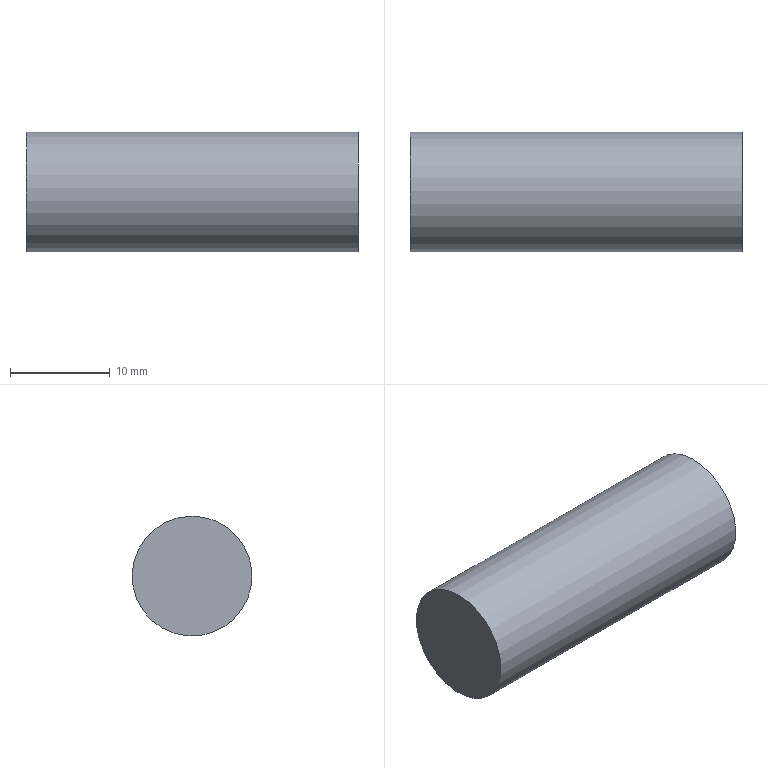Component | NX | CONNECTING_PIN | 1 solid | 3 faces | box 33.25 x 12 x 12 mm | volume 3760 mm3 | plane 2 | cylinder 1 | commonest cylinder face diameters 12 x1
STEP:
#1=CARTESIAN_POINT('',(0.,0.,0.));
#2=DIRECTION('',(0.,0.,1.));
#3=DIRECTION('',(1.,0.,0.));
#4=AXIS2_PLACEMENT_3D('',#1,#2,#3);
#5=CARTESIAN_POINT('',(-114.,-5.494,141.414));
#6=VERTEX_POINT('',#5);
#7=CARTESIAN_POINT('',(-114.,-0.25,138.498));
#8=DIRECTION('',(1.,0.,0.));
#9=DIRECTION('',(0.,-0.874,0.486));
#10=AXIS2_PLACEMENT_3D('',#7,#8,#9);
#11=CIRCLE('',#10,6.);
#12=CARTESIAN_POINT('',(-114.,-0.25,138.498));
#13=DIRECTION('',(-1.,0.,0.));
#14=DIRECTION('',(0.,-0.874,0.486));
#15=AXIS2_PLACEMENT_3D('',#12,#13,#14);
#16=PLANE('',#15);
#17=CARTESIAN_POINT('',(6.,0.));
#18=CARTESIAN_POINT('',(6.,-10.392));
#19=CARTESIAN_POINT('',(-3.,-5.196));
#20=CARTESIAN_POINT('',(-12.,-0.));
#21=CARTESIAN_POINT('',(-3.,5.196));
#22=CARTESIAN_POINT('',(6.,10.392));
#23=CARTESIAN_POINT('',(6.,0.));
#24=(BOUNDED_CURVE()B_SPLINE_CURVE(2,(#17,#18,#19,#20,#21,#22,#23),.UNSPECIFIED.,.T.,.F.)B_SPLINE_CURVE_WITH_KNOTS((1,2,2,2,2,1),(-2.094,0.,2.094,4.189,6.283,8.378),.UNSPECIFIED.)CURVE()GEOMETRIC_REPRESENTATION_ITEM()RATIONAL_B_SPLINE_CURVE((1.,0.5,1.,0.5,1.,0.5,1.))REPRESENTATION_ITEM(''));
#25=(GEOMETRIC_REPRESENTATION_CONTEXT(2)PARAMETRIC_REPRESENTATION_CONTEXT()REPRESENTATION_CONTEXT('',''));
#26=DEFINITIONAL_REPRESENTATION('',(#24),#25);
#27=PCURVE('',#16,#26);
#28=CARTESIAN_POINT('',(-80.75,-0.25,138.498));
#29=DIRECTION('',(-1.,0.,0.));
#30=DIRECTION('',(0.,-0.874,0.486));
#31=AXIS2_PLACEMENT_3D('',#28,#29,#30);
#32=CYLINDRICAL_SURFACE('',#31,6.);
#33=CARTESIAN_POINT('',(6.283,33.25));
#34=DIRECTION('',(-1.,0.));
#35=VECTOR('',#34,1.);
#36=LINE('',#33,#35);
#37=(GEOMETRIC_REPRESENTATION_CONTEXT(2)PARAMETRIC_REPRESENTATION_CONTEXT()REPRESENTATION_CONTEXT('',''));
#38=DEFINITIONAL_REPRESENTATION('',(#36),#37);
#39=PCURVE('',#32,#38);
#40=SURFACE_CURVE('',#11,(#27,#39),.PCURVE_S1.);
#41=EDGE_CURVE('',#6,#6,#40,.T.);
#42=ORIENTED_EDGE('',*,*,#41,.F.);
#43=EDGE_LOOP('',(#42));
#44=FACE_BOUND('',#43,.T.);
#45=ADVANCED_FACE('',(#44),#16,.T.);
#46=CARTESIAN_POINT('',(-80.75,-5.494,141.414));
#47=VERTEX_POINT('',#46);
#48=CARTESIAN_POINT('',(-80.75,-0.25,138.498));
#49=DIRECTION('',(-1.,0.,0.));
#50=DIRECTION('',(0.,-0.874,0.486));
#51=AXIS2_PLACEMENT_3D('',#48,#49,#50);
#52=CIRCLE('',#51,6.);
#53=CARTESIAN_POINT('',(-80.75,-0.25,138.498));
#54=DIRECTION('',(1.,0.,0.));
#55=DIRECTION('',(0.,0.874,-0.486));
#56=AXIS2_PLACEMENT_3D('',#53,#54,#55);
#57=PLANE('',#56);
#58=CARTESIAN_POINT('',(-6.,0.));
#59=CARTESIAN_POINT('',(-6.,10.392));
#60=CARTESIAN_POINT('',(3.,5.196));
#61=CARTESIAN_POINT('',(12.,-0.));
#62=CARTESIAN_POINT('',(3.,-5.196));
#63=CARTESIAN_POINT('',(-6.,-10.392));
#64=CARTESIAN_POINT('',(-6.,0.));
#65=(BOUNDED_CURVE()B_SPLINE_CURVE(2,(#58,#59,#60,#61,#62,#63,#64),.UNSPECIFIED.,.T.,.F.)B_SPLINE_CURVE_WITH_KNOTS((1,2,2,2,2,1),(-2.094,0.,2.094,4.189,6.283,8.378),.UNSPECIFIED.)CURVE()GEOMETRIC_REPRESENTATION_ITEM()RATIONAL_B_SPLINE_CURVE((1.,0.5,1.,0.5,1.,0.5,1.))REPRESENTATION_ITEM(''));
#66=(GEOMETRIC_REPRESENTATION_CONTEXT(2)PARAMETRIC_REPRESENTATION_CONTEXT()REPRESENTATION_CONTEXT('',''));
#67=DEFINITIONAL_REPRESENTATION('',(#65),#66);
#68=PCURVE('',#57,#67);
#69=CARTESIAN_POINT('',(0.,0.));
#70=DIRECTION('',(1.,0.));
#71=VECTOR('',#70,1.);
#72=LINE('',#69,#71);
#73=(GEOMETRIC_REPRESENTATION_CONTEXT(2)PARAMETRIC_REPRESENTATION_CONTEXT()REPRESENTATION_CONTEXT('',''));
#74=DEFINITIONAL_REPRESENTATION('',(#72),#73);
#75=PCURVE('',#32,#74);
#76=SURFACE_CURVE('',#52,(#68,#75),.PCURVE_S1.);
#77=EDGE_CURVE('',#47,#47,#76,.T.);
#78=ORIENTED_EDGE('',*,*,#77,.F.);
#79=EDGE_LOOP('',(#78));
#80=FACE_BOUND('',#79,.T.);
#81=ADVANCED_FACE('',(#80),#57,.T.);
#82=ORIENTED_EDGE('',*,*,#41,.T.);
#83=CARTESIAN_POINT('',(-80.75,-5.494,141.414));
#84=CARTESIAN_POINT('',(-114.,-5.494,141.414));
#85=B_SPLINE_CURVE_WITH_KNOTS('',1,(#83,#84),.UNSPECIFIED.,.F.,.F.,(2,2),(0.,33.25),.PIECEWISE_BEZIER_KNOTS.);
#86=CARTESIAN_POINT('',(0.,0.));
#87=DIRECTION('',(0.,1.));
#88=VECTOR('',#87,1.);
#89=LINE('',#86,#88);
#90=(GEOMETRIC_REPRESENTATION_CONTEXT(2)PARAMETRIC_REPRESENTATION_CONTEXT()REPRESENTATION_CONTEXT('',''));
#91=DEFINITIONAL_REPRESENTATION('',(#89),#90);
#92=PCURVE('',#32,#91);
#93=CARTESIAN_POINT('',(6.283,0.));
#94=DIRECTION('',(0.,1.));
#95=VECTOR('',#94,1.);
#96=LINE('',#93,#95);
#97=(GEOMETRIC_REPRESENTATION_CONTEXT(2)PARAMETRIC_REPRESENTATION_CONTEXT()REPRESENTATION_CONTEXT('',''));
#98=DEFINITIONAL_REPRESENTATION('',(#96),#97);
#99=PCURVE('',#32,#98);
#100=SEAM_CURVE('',#85,(#92,#99),.PCURVE_S1.);
#101=EDGE_CURVE('',#47,#6,#100,.T.);
#102=ORIENTED_EDGE('',*,*,#101,.F.);
#103=ORIENTED_EDGE('',*,*,#77,.T.);
#104=ORIENTED_EDGE('',*,*,#101,.T.);
#105=EDGE_LOOP('',(#82,#102,#103,#104));
#106=FACE_BOUND('',#105,.T.);
#107=ADVANCED_FACE('',(#106),#32,.T.);
#108=CLOSED_SHELL('',(#45,#81,#107));
#109=MANIFOLD_SOLID_BREP('',#108);
#110=(LENGTH_UNIT()NAMED_UNIT(*)SI_UNIT(.MILLI.,.METRE.));
#111=UNCERTAINTY_MEASURE_WITH_UNIT(LENGTH_MEASURE(0.00001),#110,'','');
#112=(NAMED_UNIT(*)PLANE_ANGLE_UNIT()SI_UNIT($,.RADIAN.));
#113=(NAMED_UNIT(*)SI_UNIT($,.STERADIAN.)SOLID_ANGLE_UNIT());
#114=(GEOMETRIC_REPRESENTATION_CONTEXT(3)GLOBAL_UNCERTAINTY_ASSIGNED_CONTEXT((#111))GLOBAL_UNIT_ASSIGNED_CONTEXT((#110,#112,#113))REPRESENTATION_CONTEXT('',''));
#115=ADVANCED_BREP_SHAPE_REPRESENTATION('',(#4,#109),#114);